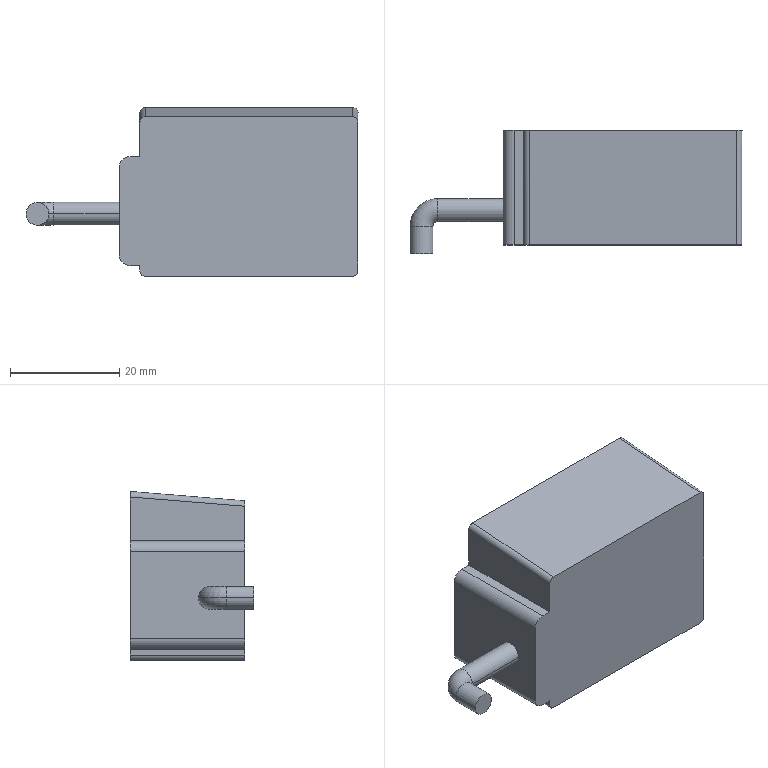Component | SolidWorks | BL-1300-2 | 1 solid | 31 faces | box 60.9 x 22.6 x 31 mm | volume 27093 mm3 | cylinder 14 | plane 11 | cone 4 | torus 2 | commonest cylinder face diameters 4.2 x4 2.5 x4 2 x4 4 x2
build123d program:
from build123d import *

# Parameters (mm, degrees)
BOSS_EXTRUDE1_DEPTH   = 20
M3_TAPPED_HOLE1_D     = 2.5
M3_TAPPED_HOLE1_DEPTH = 7.5
M3_TAPPED_HOLE1_TIP   = 0.7511
SKETCH7_W             = 20
SKETCH7_H             = 3.8
BOSS_EXTRUDE3_DEPTH   = 21
SKETCH8_R             = 2.1
FILLET1_R             = 2
FILLET2_R             = 1


with BuildPart() as part:
    # Sketch2 → Boss-Extrude1 (new, symmetric)
    with BuildSketch(Plane.XY):
        Polygon((0, 0), (31, 0), (29.3, 21), (0, 21), align=None)
    extrude(amount=BOSS_EXTRUDE1_DEPTH, both=True)

    # M3 Tapped Hole1
    with Locations(Plane(origin=(0, 0, 0), x_dir=(-1, 0, 0), z_dir=(0, -1, 0))):
        with Locations((-3.5, -16.5), (-26, 16.5)):
            Hole(M3_TAPPED_HOLE1_D / 2, depth=M3_TAPPED_HOLE1_DEPTH)
            with Locations((0, 0, -(M3_TAPPED_HOLE1_DEPTH + M3_TAPPED_HOLE1_TIP / 2))):  # 118° drill point
                Cone(0, M3_TAPPED_HOLE1_D / 2, M3_TAPPED_HOLE1_TIP, mode=Mode.SUBTRACT)

    # Sketch7 → Boss-Extrude3 (add)
    with BuildSketch(Plane.XZ):
        with Locations((12, -21.9)):
            Rectangle(SKETCH7_W, SKETCH7_H)
    extrude(amount=-BOSS_EXTRUDE3_DEPTH)

    # Sweep1: sweep along a path in Sketch9
    with BuildLine(Plane.ZY.offset(-11.5)) as sweep1_path:
        Line((-23.8, 14.6), (-35.8, 14.6))
        ThreePointArc((-35.8, 14.6), (-37.921, 15.479), (-38.8, 17.6))
        Line((-38.8, 17.6), (-38.8, 22.6))
    # Sketch8 → Sweep1 (sweep)
    with BuildSketch(Plane(origin=(0, 0, -23.8), x_dir=(-1, 0, 0), z_dir=(0, 0, -1))):
        with Locations((-11.5, 14.6)):
            Circle(SKETCH8_R)
    sweep(path=sweep1_path.line)

    # Fillet1
    fillet1_edges = [part.edges().sort_by_distance(p)[0] for p in [
        (22, 10.5, -23.8),
        (2, 10.5, -23.8),
    ]]
    fillet(fillet1_edges, radius=FILLET1_R)

    # Fillet2
    fillet2_edges = [part.edges().sort_by_distance(p)[0] for p in [
        (30.15, 10.5, 20),
        (30.15, 10.5, -20),
        (0, 10.5, -20),
        (0, 10.5, 20),
    ]]
    fillet(fillet2_edges, radius=FILLET2_R)


solid = part.part

# Placed as in the assembly
solid = solid.moved(Location((-14.281, -110.523, -276.479), (180, 90, 0)))
STEP:
#1=CARTESIAN_POINT('',(-1.972,-5.009,-10.432));
#2=VERTEX_POINT('',#1);
#3=CARTESIAN_POINT('',(-1.972,-4.843,-10.432));
#4=VERTEX_POINT('',#3);
#5=CARTESIAN_POINT('',(-1.972,-4.926,-10.432));
#6=DIRECTION('',(-1.,-0.,0.));
#7=DIRECTION('',(-0.,0.,-1.));
#8=AXIS2_PLACEMENT_3D('',#5,#6,#7);
#9=CIRCLE('',#8,0.08268);
#10=EDGE_CURVE('',#2,#4,#9,.T.);
#11=ORIENTED_EDGE('',*,*,#10,.T.);
#12=CARTESIAN_POINT('',(-2.172,-5.044,-10.432));
#13=VERTEX_POINT('',#12);
#14=CARTESIAN_POINT('',(-1.972,-5.044,-10.432));
#15=DIRECTION('',(0.,0.,1.));
#16=DIRECTION('',(1.,0.,-0.));
#17=AXIS2_PLACEMENT_3D('',#14,#15,#16);
#18=CIRCLE('',#17,0.2008);
#19=EDGE_CURVE('',#4,#13,#18,.T.);
#20=ORIENTED_EDGE('',*,*,#19,.T.);
#21=CARTESIAN_POINT('',(-2.007,-5.044,-10.432));
#22=VERTEX_POINT('',#21);
#23=CARTESIAN_POINT('',(-2.09,-5.044,-10.432));
#24=DIRECTION('',(0.,-1.,0.));
#25=DIRECTION('',(-0.,0.,-1.));
#26=AXIS2_PLACEMENT_3D('',#23,#24,#25);
#27=CIRCLE('',#26,0.08268);
#28=EDGE_CURVE('',#22,#13,#27,.T.);
#29=ORIENTED_EDGE('',*,*,#28,.F.);
#30=CARTESIAN_POINT('',(-1.972,-5.044,-10.432));
#31=DIRECTION('',(0.,0.,1.));
#32=DIRECTION('',(1.,0.,-0.));
#33=AXIS2_PLACEMENT_3D('',#30,#31,#32);
#34=CIRCLE('',#33,0.03543);
#35=EDGE_CURVE('',#2,#22,#34,.T.);
#36=ORIENTED_EDGE('',*,*,#35,.F.);
#37=EDGE_LOOP('',(#11,#20,#29,#36));
#38=FACE_OUTER_BOUND('',#37,.T.);
#39=CARTESIAN_POINT('',(-1.972,-5.044,-10.432));
#40=DIRECTION('',(0.,0.,1.));
#41=DIRECTION('',(0.,-1.,0.));
#42=AXIS2_PLACEMENT_3D('',#39,#40,#41);
#43=TOROIDAL_SURFACE('',#42,0.1181,0.08268);
#44=ADVANCED_FACE('',(#38),#43,.T.);
#45=ORIENTED_EDGE('',*,*,#10,.F.);
#46=CARTESIAN_POINT('',(-1.499,-5.009,-10.432));
#47=VERTEX_POINT('',#46);
#48=CARTESIAN_POINT('',(-1.972,-5.009,-10.432));
#49=DIRECTION('',(1.,0.,-0.));
#50=VECTOR('',#49,39.37);
#51=LINE('',#48,#50);
#52=EDGE_CURVE('',#2,#47,#51,.T.);
#53=ORIENTED_EDGE('',*,*,#52,.T.);
#54=CARTESIAN_POINT('',(-1.499,-4.843,-10.432));
#55=VERTEX_POINT('',#54);
#56=CARTESIAN_POINT('',(-1.499,-4.926,-10.432));
#57=DIRECTION('',(-1.,-0.,0.));
#58=DIRECTION('',(-0.,0.,-1.));
#59=AXIS2_PLACEMENT_3D('',#56,#57,#58);
#60=CIRCLE('',#59,0.08268);
#61=EDGE_CURVE('',#47,#55,#60,.T.);
#62=ORIENTED_EDGE('',*,*,#61,.T.);
#63=CARTESIAN_POINT('',(-1.972,-4.843,-10.432));
#64=DIRECTION('',(1.,0.,-0.));
#65=VECTOR('',#64,39.37);
#66=LINE('',#63,#65);
#67=EDGE_CURVE('',#4,#55,#66,.T.);
#68=ORIENTED_EDGE('',*,*,#67,.F.);
#69=EDGE_LOOP('',(#45,#53,#62,#68));
#70=FACE_OUTER_BOUND('',#69,.T.);
#71=CARTESIAN_POINT('',(-1.972,-4.926,-10.432));
#72=DIRECTION('',(1.,0.,-0.));
#73=DIRECTION('',(0.,1.,0.));
#74=AXIS2_PLACEMENT_3D('',#71,#72,#73);
#75=CYLINDRICAL_SURFACE('',#74,0.08268);
#76=ADVANCED_FACE('',(#70),#75,.T.);
#77=ORIENTED_EDGE('',*,*,#28,.T.);
#78=CARTESIAN_POINT('',(-2.172,-5.241,-10.432));
#79=VERTEX_POINT('',#78);
#80=CARTESIAN_POINT('',(-2.172,-5.044,-10.432));
#81=DIRECTION('',(0.,-1.,0.));
#82=VECTOR('',#81,39.37);
#83=LINE('',#80,#82);
#84=EDGE_CURVE('',#13,#79,#83,.T.);
#85=ORIENTED_EDGE('',*,*,#84,.T.);
#86=CARTESIAN_POINT('',(-2.007,-5.241,-10.432));
#87=VERTEX_POINT('',#86);
#88=CARTESIAN_POINT('',(-2.09,-5.241,-10.432));
#89=DIRECTION('',(0.,-1.,0.));
#90=DIRECTION('',(-0.,0.,-1.));
#91=AXIS2_PLACEMENT_3D('',#88,#89,#90);
#92=CIRCLE('',#91,0.08268);
#93=EDGE_CURVE('',#87,#79,#92,.T.);
#94=ORIENTED_EDGE('',*,*,#93,.F.);
#95=CARTESIAN_POINT('',(-2.007,-5.044,-10.432));
#96=DIRECTION('',(0.,-1.,0.));
#97=VECTOR('',#96,39.37);
#98=LINE('',#95,#97);
#99=EDGE_CURVE('',#22,#87,#98,.T.);
#100=ORIENTED_EDGE('',*,*,#99,.F.);
#101=EDGE_LOOP('',(#77,#85,#94,#100));
#102=FACE_OUTER_BOUND('',#101,.T.);
#103=CARTESIAN_POINT('',(-2.09,-5.044,-10.432));
#104=DIRECTION('',(0.,-1.,0.));
#105=DIRECTION('',(1.,0.,-0.));
#106=AXIS2_PLACEMENT_3D('',#103,#104,#105);
#107=CYLINDRICAL_SURFACE('',#106,0.08268);
#108=ADVANCED_FACE('',(#102),#107,.T.);
#109=CARTESIAN_POINT('',(0.1366,-4.647,-10.747));
#110=VERTEX_POINT('',#109);
#111=CARTESIAN_POINT('',(0.03816,-4.647,-10.747));
#112=VERTEX_POINT('',#111);
#113=CARTESIAN_POINT('',(0.08738,-4.647,-10.747));
#114=DIRECTION('',(-0.,1.,-0.));
#115=DIRECTION('',(-1.,0.,0.));
#116=AXIS2_PLACEMENT_3D('',#113,#114,#115);
#117=CIRCLE('',#116,0.04921);
#118=EDGE_CURVE('',#110,#112,#117,.T.);
#119=ORIENTED_EDGE('',*,*,#118,.F.);
#120=CARTESIAN_POINT('',(0.1366,-4.351,-10.747));
#121=VERTEX_POINT('',#120);
#122=CARTESIAN_POINT('',(0.1366,-4.351,-10.747));
#123=DIRECTION('',(-0.,1.,-0.));
#124=VECTOR('',#123,39.37);
#125=LINE('',#122,#124);
#126=EDGE_CURVE('',#110,#121,#125,.T.);
#127=ORIENTED_EDGE('',*,*,#126,.T.);
#128=CARTESIAN_POINT('',(0.03816,-4.351,-10.747));
#129=VERTEX_POINT('',#128);
#130=CARTESIAN_POINT('',(0.08738,-4.351,-10.747));
#131=DIRECTION('',(-0.,1.,-0.));
#132=DIRECTION('',(-1.,0.,0.));
#133=AXIS2_PLACEMENT_3D('',#130,#131,#132);
#134=CIRCLE('',#133,0.04921);
#135=EDGE_CURVE('',#121,#129,#134,.T.);
#136=ORIENTED_EDGE('',*,*,#135,.T.);
#137=CARTESIAN_POINT('',(0.03816,-4.351,-10.747));
#138=DIRECTION('',(-0.,1.,-0.));
#139=VECTOR('',#138,39.37);
#140=LINE('',#137,#139);
#141=EDGE_CURVE('',#112,#129,#140,.T.);
#142=ORIENTED_EDGE('',*,*,#141,.F.);
#143=EDGE_LOOP('',(#119,#127,#136,#142));
#144=FACE_OUTER_BOUND('',#143,.T.);
#145=CARTESIAN_POINT('',(0.08738,-4.351,-10.747));
#146=DIRECTION('',(-0.,1.,-0.));
#147=DIRECTION('',(-1.,0.,0.));
#148=AXIS2_PLACEMENT_3D('',#145,#146,#147);
#149=CYLINDRICAL_SURFACE('',#148,0.04921);
#150=ADVANCED_FACE('',(#144),#149,.F.);
#151=CARTESIAN_POINT('',(0.08738,-4.676,-10.747));
#152=VERTEX_POINT('',#151);
#153=CARTESIAN_POINT('',(0.03816,-4.647,-10.747));
#154=DIRECTION('',(-0.8572,0.515,0.));
#155=VECTOR('',#154,39.37);
#156=LINE('',#153,#155);
#157=EDGE_CURVE('',#152,#112,#156,.T.);
#158=ORIENTED_EDGE('',*,*,#157,.F.);
#159=CARTESIAN_POINT('',(0.1366,-4.647,-10.747));
#160=DIRECTION('',(0.8572,0.515,-0.));
#161=VECTOR('',#160,39.37);
#162=LINE('',#159,#161);
#163=EDGE_CURVE('',#152,#110,#162,.T.);
#164=ORIENTED_EDGE('',*,*,#163,.T.);
#165=ORIENTED_EDGE('',*,*,#118,.T.);
#166=EDGE_LOOP('',(#158,#164,#165));
#167=FACE_OUTER_BOUND('',#166,.T.);
#168=CARTESIAN_POINT('',(0.08738,-4.647,-10.747));
#169=DIRECTION('',(-0.,1.,-0.));
#170=DIRECTION('',(-1.,0.,0.));
#171=AXIS2_PLACEMENT_3D('',#168,#169,#170);
#172=CONICAL_SURFACE('',#171,0.04921,1.03);
#173=ADVANCED_FACE('',(#167),#172,.F.);
#174=CARTESIAN_POINT('',(-1.163,-4.647,-9.861));
#175=VERTEX_POINT('',#174);
#176=CARTESIAN_POINT('',(-1.261,-4.647,-9.861));
#177=VERTEX_POINT('',#176);
#178=CARTESIAN_POINT('',(-1.212,-4.647,-9.861));
#179=DIRECTION('',(-0.,1.,-0.));
#180=DIRECTION('',(-1.,0.,0.));
#181=AXIS2_PLACEMENT_3D('',#178,#179,#180);
#182=CIRCLE('',#181,0.04921);
#183=EDGE_CURVE('',#175,#177,#182,.T.);
#184=ORIENTED_EDGE('',*,*,#183,.F.);
#185=CARTESIAN_POINT('',(-1.163,-4.351,-9.861));
#186=VERTEX_POINT('',#185);
#187=CARTESIAN_POINT('',(-1.163,-4.351,-9.861));
#188=DIRECTION('',(-0.,1.,-0.));
#189=VECTOR('',#188,39.37);
#190=LINE('',#187,#189);
#191=EDGE_CURVE('',#175,#186,#190,.T.);
#192=ORIENTED_EDGE('',*,*,#191,.T.);
#193=CARTESIAN_POINT('',(-1.261,-4.351,-9.861));
#194=VERTEX_POINT('',#193);
#195=CARTESIAN_POINT('',(-1.212,-4.351,-9.861));
#196=DIRECTION('',(-0.,1.,-0.));
#197=DIRECTION('',(-1.,0.,0.));
#198=AXIS2_PLACEMENT_3D('',#195,#196,#197);
#199=CIRCLE('',#198,0.04921);
#200=EDGE_CURVE('',#186,#194,#199,.T.);
#201=ORIENTED_EDGE('',*,*,#200,.T.);
#202=CARTESIAN_POINT('',(-1.261,-4.351,-9.861));
#203=DIRECTION('',(-0.,1.,-0.));
#204=VECTOR('',#203,39.37);
#205=LINE('',#202,#204);
#206=EDGE_CURVE('',#177,#194,#205,.T.);
#207=ORIENTED_EDGE('',*,*,#206,.F.);
#208=EDGE_LOOP('',(#184,#192,#201,#207));
#209=FACE_OUTER_BOUND('',#208,.T.);
#210=CARTESIAN_POINT('',(-1.212,-4.351,-9.861));
#211=DIRECTION('',(-0.,1.,-0.));
#212=DIRECTION('',(-1.,0.,0.));
#213=AXIS2_PLACEMENT_3D('',#210,#211,#212);
#214=CYLINDRICAL_SURFACE('',#213,0.04921);
#215=ADVANCED_FACE('',(#209),#214,.F.);
#216=CARTESIAN_POINT('',(-1.212,-4.676,-9.861));
#217=VERTEX_POINT('',#216);
#218=CARTESIAN_POINT('',(-1.261,-4.647,-9.861));
#219=DIRECTION('',(-0.8572,0.515,0.));
#220=VECTOR('',#219,39.37);
#221=LINE('',#218,#220);
#222=EDGE_CURVE('',#217,#177,#221,.T.);
#223=ORIENTED_EDGE('',*,*,#222,.F.);
#224=CARTESIAN_POINT('',(-1.163,-4.647,-9.861));
#225=DIRECTION('',(0.8572,0.515,-0.));
#226=VECTOR('',#225,39.37);
#227=LINE('',#224,#226);
#228=EDGE_CURVE('',#217,#175,#227,.T.);
#229=ORIENTED_EDGE('',*,*,#228,.T.);
#230=ORIENTED_EDGE('',*,*,#183,.T.);
#231=EDGE_LOOP('',(#223,#229,#230));
#232=FACE_OUTER_BOUND('',#231,.T.);
#233=CARTESIAN_POINT('',(-1.212,-4.647,-9.861));
#234=DIRECTION('',(-0.,1.,-0.));
#235=DIRECTION('',(-1.,0.,0.));
#236=AXIS2_PLACEMENT_3D('',#233,#234,#235);
#237=CONICAL_SURFACE('',#236,0.04921,1.03);
#238=ADVANCED_FACE('',(#232),#237,.F.);
#239=CARTESIAN_POINT('',(-1.35,-5.178,-9.771));
#240=VERTEX_POINT('',#239);
#241=CARTESIAN_POINT('',(-1.35,-5.178,-10.019));
#242=VERTEX_POINT('',#241);
#243=CARTESIAN_POINT('',(-1.35,-5.178,-9.731));
#244=DIRECTION('',(-0.,-0.,-1.));
#245=VECTOR('',#244,39.37);
#246=LINE('',#243,#245);
#247=EDGE_CURVE('',#240,#242,#246,.T.);
#248=ORIENTED_EDGE('',*,*,#247,.F.);
#249=CARTESIAN_POINT('',(-1.35,-4.351,-9.704));
#250=VERTEX_POINT('',#249);
#251=CARTESIAN_POINT('',(-1.35,-4.446,-9.712));
#252=DIRECTION('',(0.,0.9967,0.08069));
#253=VECTOR('',#252,39.37);
#254=LINE('',#251,#253);
#255=EDGE_CURVE('',#240,#250,#254,.T.);
#256=ORIENTED_EDGE('',*,*,#255,.T.);
#257=CARTESIAN_POINT('',(-1.35,-4.351,-10.019));
#258=VERTEX_POINT('',#257);
#259=CARTESIAN_POINT('',(-1.35,-4.351,-10.885));
#260=DIRECTION('',(0.,0.,1.));
#261=VECTOR('',#260,39.37);
#262=LINE('',#259,#261);
#263=EDGE_CURVE('',#258,#250,#262,.T.);
#264=ORIENTED_EDGE('',*,*,#263,.F.);
#265=CARTESIAN_POINT('',(-1.35,-5.98,-10.019));
#266=DIRECTION('',(-0.,1.,-0.));
#267=VECTOR('',#266,39.37);
#268=LINE('',#265,#267);
#269=EDGE_CURVE('',#242,#258,#268,.T.);
#270=ORIENTED_EDGE('',*,*,#269,.F.);
#271=EDGE_LOOP('',(#248,#256,#264,#270));
#272=FACE_OUTER_BOUND('',#271,.T.);
#273=CARTESIAN_POINT('',(-1.35,-4.351,-10.885));
#274=DIRECTION('',(1.,0.,-0.));
#275=DIRECTION('',(0.,0.,1.));
#276=AXIS2_PLACEMENT_3D('',#273,#274,#275);
#277=PLANE('',#276);
#278=ADVANCED_FACE('',(#272),#277,.F.);
#279=CARTESIAN_POINT('',(0.1858,-5.178,-10.885));
#280=VERTEX_POINT('',#279);
#281=CARTESIAN_POINT('',(-1.31,-5.178,-10.885));
#282=VERTEX_POINT('',#281);
#283=CARTESIAN_POINT('',(0.2252,-5.178,-10.885));
#284=DIRECTION('',(-1.,-0.,0.));
#285=VECTOR('',#284,39.37);
#286=LINE('',#283,#285);
#287=EDGE_CURVE('',#280,#282,#286,.T.);
#288=ORIENTED_EDGE('',*,*,#287,.T.);
#289=CARTESIAN_POINT('',(-1.31,-4.351,-10.885));
#290=VERTEX_POINT('',#289);
#291=CARTESIAN_POINT('',(-1.31,-5.178,-10.885));
#292=DIRECTION('',(-0.,1.,-0.));
#293=VECTOR('',#292,39.37);
#294=LINE('',#291,#293);
#295=EDGE_CURVE('',#282,#290,#294,.T.);
#296=ORIENTED_EDGE('',*,*,#295,.T.);
#297=CARTESIAN_POINT('',(0.1858,-4.351,-10.885));
#298=VERTEX_POINT('',#297);
#299=CARTESIAN_POINT('',(0.2252,-4.351,-10.885));
#300=DIRECTION('',(-1.,-0.,0.));
#301=VECTOR('',#300,39.37);
#302=LINE('',#299,#301);
#303=EDGE_CURVE('',#298,#290,#302,.T.);
#304=ORIENTED_EDGE('',*,*,#303,.F.);
#305=CARTESIAN_POINT('',(0.1858,-5.178,-10.885));
#306=DIRECTION('',(0.,-1.,0.));
#307=VECTOR('',#306,39.37);
#308=LINE('',#305,#307);
#309=EDGE_CURVE('',#298,#280,#308,.T.);
#310=ORIENTED_EDGE('',*,*,#309,.T.);
#311=EDGE_LOOP('',(#288,#296,#304,#310));
#312=FACE_OUTER_BOUND('',#311,.T.);
#313=CARTESIAN_POINT('',(0.2252,-5.178,-10.885));
#314=DIRECTION('',(0.,0.,1.));
#315=DIRECTION('',(0.,-1.,0.));
#316=AXIS2_PLACEMENT_3D('',#313,#314,#315);
#317=PLANE('',#316);
#318=ADVANCED_FACE('',(#312),#317,.F.);
#319=CARTESIAN_POINT('',(0.08738,-4.351,-10.747));
#320=DIRECTION('',(-0.,1.,-0.));
#321=DIRECTION('',(-1.,0.,0.));
#322=AXIS2_PLACEMENT_3D('',#319,#320,#321);
#323=CIRCLE('',#322,0.04921);
#324=EDGE_CURVE('',#129,#121,#323,.T.);
#325=ORIENTED_EDGE('',*,*,#324,.F.);
#326=ORIENTED_EDGE('',*,*,#135,.F.);
#327=EDGE_LOOP('',(#325,#326));
#328=FACE_BOUND('',#327,.T.);
#329=CARTESIAN_POINT('',(-1.212,-4.351,-9.861));
#330=DIRECTION('',(-0.,1.,-0.));
#331=DIRECTION('',(-1.,0.,0.));
#332=AXIS2_PLACEMENT_3D('',#329,#330,#331);
#333=CIRCLE('',#332,0.04921);
#334=EDGE_CURVE('',#194,#186,#333,.T.);
#335=ORIENTED_EDGE('',*,*,#334,.F.);
#336=ORIENTED_EDGE('',*,*,#200,.F.);
#337=EDGE_LOOP('',(#335,#336));
#338=FACE_BOUND('',#337,.T.);
#339=ORIENTED_EDGE('',*,*,#263,.T.);
#340=CARTESIAN_POINT('',(-1.31,-4.351,-9.665));
#341=VERTEX_POINT('',#340);
#342=CARTESIAN_POINT('',(-1.35,-4.351,-9.704));
#343=CARTESIAN_POINT('',(-1.35,-4.351,-9.681));
#344=CARTESIAN_POINT('',(-1.333,-4.351,-9.665));
#345=CARTESIAN_POINT('',(-1.31,-4.351,-9.665));
#346=(BOUNDED_CURVE()B_SPLINE_CURVE(3,(#342,#343,#344,#345),.UNSPECIFIED.,.F.,.T.)B_SPLINE_CURVE_WITH_KNOTS((4,4),(1.571,3.142),.UNSPECIFIED.)CURVE()GEOMETRIC_REPRESENTATION_ITEM()RATIONAL_B_SPLINE_CURVE((1.,0.8047,0.8047,1.))REPRESENTATION_ITEM(''));
#347=EDGE_CURVE('',#250,#341,#346,.T.);
#348=ORIENTED_EDGE('',*,*,#347,.T.);
#349=CARTESIAN_POINT('',(0.1858,-4.351,-9.665));
#350=VERTEX_POINT('',#349);
#351=CARTESIAN_POINT('',(0.2252,-4.351,-9.665));
#352=DIRECTION('',(-1.,-0.,0.));
#353=VECTOR('',#352,39.37);
#354=LINE('',#351,#353);
#355=EDGE_CURVE('',#350,#341,#354,.T.);
#356=ORIENTED_EDGE('',*,*,#355,.F.);
#357=CARTESIAN_POINT('',(0.2252,-4.351,-9.704));
#358=VERTEX_POINT('',#357);
#359=CARTESIAN_POINT('',(0.1858,-4.351,-9.665));
#360=CARTESIAN_POINT('',(0.2089,-4.351,-9.665));
#361=CARTESIAN_POINT('',(0.2252,-4.351,-9.681));
#362=CARTESIAN_POINT('',(0.2252,-4.351,-9.704));
#363=(BOUNDED_CURVE()B_SPLINE_CURVE(3,(#359,#360,#361,#362),.UNSPECIFIED.,.F.,.T.)B_SPLINE_CURVE_WITH_KNOTS((4,4),(0.,1.571),.UNSPECIFIED.)CURVE()GEOMETRIC_REPRESENTATION_ITEM()RATIONAL_B_SPLINE_CURVE((1.,0.8047,0.8047,1.))REPRESENTATION_ITEM(''));
#364=EDGE_CURVE('',#350,#358,#363,.T.);
#365=ORIENTED_EDGE('',*,*,#364,.T.);
#366=CARTESIAN_POINT('',(0.2252,-4.351,-10.846));
#367=VERTEX_POINT('',#366);
#368=CARTESIAN_POINT('',(0.2252,-4.351,-10.885));
#369=DIRECTION('',(0.,0.,1.));
#370=VECTOR('',#369,39.37);
#371=LINE('',#368,#370);
#372=EDGE_CURVE('',#367,#358,#371,.T.);
#373=ORIENTED_EDGE('',*,*,#372,.F.);
#374=CARTESIAN_POINT('',(0.1858,-4.351,-10.846));
#375=DIRECTION('',(-0.,1.,-0.));
#376=DIRECTION('',(1.,0.,-0.));
#377=AXIS2_PLACEMENT_3D('',#374,#375,#376);
#378=CIRCLE('',#377,0.03937);
#379=EDGE_CURVE('',#367,#298,#378,.T.);
#380=ORIENTED_EDGE('',*,*,#379,.T.);
#381=ORIENTED_EDGE('',*,*,#303,.T.);
#382=CARTESIAN_POINT('',(-1.35,-4.351,-10.846));
#383=VERTEX_POINT('',#382);
#384=CARTESIAN_POINT('',(-1.31,-4.351,-10.846));
#385=DIRECTION('',(-0.,1.,-0.));
#386=DIRECTION('',(1.,0.,-0.));
#387=AXIS2_PLACEMENT_3D('',#384,#385,#386);
#388=CIRCLE('',#387,0.03937);
#389=EDGE_CURVE('',#290,#383,#388,.T.);
#390=ORIENTED_EDGE('',*,*,#389,.T.);
#391=CARTESIAN_POINT('',(-1.35,-4.351,-10.806));
#392=VERTEX_POINT('',#391);
#393=CARTESIAN_POINT('',(-1.35,-4.351,-10.885));
#394=DIRECTION('',(0.,0.,1.));
#395=VECTOR('',#394,39.37);
#396=LINE('',#393,#395);
#397=EDGE_CURVE('',#383,#392,#396,.T.);
#398=ORIENTED_EDGE('',*,*,#397,.T.);
#399=CARTESIAN_POINT('',(-1.42,-4.351,-10.806));
#400=VERTEX_POINT('',#399);
#401=CARTESIAN_POINT('',(-1.35,-4.351,-10.806));
#402=DIRECTION('',(-1.,-0.,0.));
#403=VECTOR('',#402,39.37);
#404=LINE('',#401,#403);
#405=EDGE_CURVE('',#392,#400,#404,.T.);
#406=ORIENTED_EDGE('',*,*,#405,.T.);
#407=CARTESIAN_POINT('',(-1.499,-4.351,-10.728));
#408=VERTEX_POINT('',#407);
#409=CARTESIAN_POINT('',(-1.42,-4.351,-10.728));
#410=DIRECTION('',(-0.,1.,-0.));
#411=DIRECTION('',(1.,0.,-0.));
#412=AXIS2_PLACEMENT_3D('',#409,#410,#411);
#413=CIRCLE('',#412,0.07874);
#414=EDGE_CURVE('',#400,#408,#413,.T.);
#415=ORIENTED_EDGE('',*,*,#414,.T.);
#416=CARTESIAN_POINT('',(-1.499,-4.351,-10.098));
#417=VERTEX_POINT('',#416);
#418=CARTESIAN_POINT('',(-1.499,-4.351,-10.806));
#419=DIRECTION('',(0.,0.,1.));
#420=VECTOR('',#419,39.37);
#421=LINE('',#418,#420);
#422=EDGE_CURVE('',#408,#417,#421,.T.);
#423=ORIENTED_EDGE('',*,*,#422,.T.);
#424=CARTESIAN_POINT('',(-1.42,-4.351,-10.019));
#425=VERTEX_POINT('',#424);
#426=CARTESIAN_POINT('',(-1.42,-4.351,-10.098));
#427=DIRECTION('',(-0.,1.,-0.));
#428=DIRECTION('',(1.,0.,-0.));
#429=AXIS2_PLACEMENT_3D('',#426,#427,#428);
#430=CIRCLE('',#429,0.07874);
#431=EDGE_CURVE('',#417,#425,#430,.T.);
#432=ORIENTED_EDGE('',*,*,#431,.T.);
#433=CARTESIAN_POINT('',(-1.35,-4.351,-10.019));
#434=DIRECTION('',(1.,0.,-0.));
#435=VECTOR('',#434,39.37);
#436=LINE('',#433,#435);
#437=EDGE_CURVE('',#425,#258,#436,.T.);
#438=ORIENTED_EDGE('',*,*,#437,.T.);
#439=EDGE_LOOP('',(#339,#348,#356,#365,#373,#380,#381,#390,#398,#406,#415,#423,#432,#438));
#440=FACE_OUTER_BOUND('',#439,.T.);
#441=CARTESIAN_POINT('',(0.2252,-4.351,-10.885));
#442=DIRECTION('',(0.,-1.,0.));
#443=DIRECTION('',(1.,0.,-0.));
#444=AXIS2_PLACEMENT_3D('',#441,#442,#443);
#445=PLANE('',#444);
#446=ADVANCED_FACE('',(#328,#338,#440),#445,.F.);
#447=ORIENTED_EDGE('',*,*,#355,.T.);
#448=CARTESIAN_POINT('',(-1.31,-5.178,-9.731));
#449=VERTEX_POINT('',#448);
#450=CARTESIAN_POINT('',(-1.31,-4.351,-9.665));
#451=DIRECTION('',(-0.,-0.9967,-0.08069));
#452=VECTOR('',#451,39.37);
#453=LINE('',#450,#452);
#454=EDGE_CURVE('',#341,#449,#453,.T.);
#455=ORIENTED_EDGE('',*,*,#454,.T.);
#456=CARTESIAN_POINT('',(0.1858,-5.178,-9.731));
#457=VERTEX_POINT('',#456);
#458=CARTESIAN_POINT('',(0.2252,-5.178,-9.731));
#459=DIRECTION('',(-1.,-0.,0.));
#460=VECTOR('',#459,39.37);
#461=LINE('',#458,#460);
#462=EDGE_CURVE('',#457,#449,#461,.T.);
#463=ORIENTED_EDGE('',*,*,#462,.F.);
#464=CARTESIAN_POINT('',(0.1858,-4.351,-9.665));
#465=DIRECTION('',(0.,0.9967,0.08069));
#466=VECTOR('',#465,39.37);
#467=LINE('',#464,#466);
#468=EDGE_CURVE('',#457,#350,#467,.T.);
#469=ORIENTED_EDGE('',*,*,#468,.T.);
#470=EDGE_LOOP('',(#447,#455,#463,#469));
#471=FACE_OUTER_BOUND('',#470,.T.);
#472=CARTESIAN_POINT('',(0.2252,-4.351,-9.665));
#473=DIRECTION('',(-0.,0.08069,-0.9967));
#474=DIRECTION('',(0.,0.9967,0.08069));
#475=AXIS2_PLACEMENT_3D('',#472,#473,#474);
#476=PLANE('',#475);
#477=ADVANCED_FACE('',(#471),#476,.F.);
#478=ORIENTED_EDGE('',*,*,#462,.T.);
#479=CARTESIAN_POINT('',(-1.31,-5.178,-9.731));
#480=CARTESIAN_POINT('',(-1.333,-5.178,-9.731));
#481=CARTESIAN_POINT('',(-1.35,-5.178,-9.748));
#482=CARTESIAN_POINT('',(-1.35,-5.178,-9.771));
#483=(BOUNDED_CURVE()B_SPLINE_CURVE(3,(#479,#480,#481,#482),.UNSPECIFIED.,.F.,.T.)B_SPLINE_CURVE_WITH_KNOTS((4,4),(3.142,4.712),.UNSPECIFIED.)CURVE()GEOMETRIC_REPRESENTATION_ITEM()RATIONAL_B_SPLINE_CURVE((1.,0.8047,0.8047,1.))REPRESENTATION_ITEM(''));
#484=EDGE_CURVE('',#449,#240,#483,.T.);
#485=ORIENTED_EDGE('',*,*,#484,.T.);
#486=ORIENTED_EDGE('',*,*,#247,.T.);
#487=CARTESIAN_POINT('',(-1.42,-5.178,-10.019));
#488=VERTEX_POINT('',#487);
#489=CARTESIAN_POINT('',(-1.35,-5.178,-10.019));
#490=DIRECTION('',(-1.,-0.,0.));
#491=VECTOR('',#490,39.37);
#492=LINE('',#489,#491);
#493=EDGE_CURVE('',#242,#488,#492,.T.);
#494=ORIENTED_EDGE('',*,*,#493,.T.);
#495=CARTESIAN_POINT('',(-1.499,-5.178,-10.098));
#496=VERTEX_POINT('',#495);
#497=CARTESIAN_POINT('',(-1.42,-5.178,-10.098));
#498=DIRECTION('',(0.,-1.,0.));
#499=DIRECTION('',(0.,0.,1.));
#500=AXIS2_PLACEMENT_3D('',#497,#498,#499);
#501=CIRCLE('',#500,0.07874);
#502=EDGE_CURVE('',#488,#496,#501,.T.);
#503=ORIENTED_EDGE('',*,*,#502,.T.);
#504=CARTESIAN_POINT('',(-1.499,-5.178,-10.728));
#505=VERTEX_POINT('',#504);
#506=CARTESIAN_POINT('',(-1.499,-5.178,-10.806));
#507=DIRECTION('',(-0.,-0.,-1.));
#508=VECTOR('',#507,39.37);
#509=LINE('',#506,#508);
#510=EDGE_CURVE('',#496,#505,#509,.T.);
#511=ORIENTED_EDGE('',*,*,#510,.T.);
#512=CARTESIAN_POINT('',(-1.42,-5.178,-10.806));
#513=VERTEX_POINT('',#512);
#514=CARTESIAN_POINT('',(-1.42,-5.178,-10.728));
#515=DIRECTION('',(0.,-1.,0.));
#516=DIRECTION('',(0.,0.,1.));
#517=AXIS2_PLACEMENT_3D('',#514,#515,#516);
#518=CIRCLE('',#517,0.07874);
#519=EDGE_CURVE('',#505,#513,#518,.T.);
#520=ORIENTED_EDGE('',*,*,#519,.T.);
#521=CARTESIAN_POINT('',(-1.35,-5.178,-10.806));
#522=VERTEX_POINT('',#521);
#523=CARTESIAN_POINT('',(-1.35,-5.178,-10.806));
#524=DIRECTION('',(1.,0.,-0.));
#525=VECTOR('',#524,39.37);
#526=LINE('',#523,#525);
#527=EDGE_CURVE('',#513,#522,#526,.T.);
#528=ORIENTED_EDGE('',*,*,#527,.T.);
#529=CARTESIAN_POINT('',(-1.35,-5.178,-10.846));
#530=VERTEX_POINT('',#529);
#531=CARTESIAN_POINT('',(-1.35,-5.178,-9.731));
#532=DIRECTION('',(-0.,-0.,-1.));
#533=VECTOR('',#532,39.37);
#534=LINE('',#531,#533);
#535=EDGE_CURVE('',#522,#530,#534,.T.);
#536=ORIENTED_EDGE('',*,*,#535,.T.);
#537=CARTESIAN_POINT('',(-1.31,-5.178,-10.846));
#538=DIRECTION('',(0.,-1.,0.));
#539=DIRECTION('',(0.,0.,1.));
#540=AXIS2_PLACEMENT_3D('',#537,#538,#539);
#541=CIRCLE('',#540,0.03937);
#542=EDGE_CURVE('',#530,#282,#541,.T.);
#543=ORIENTED_EDGE('',*,*,#542,.T.);
#544=ORIENTED_EDGE('',*,*,#287,.F.);
#545=CARTESIAN_POINT('',(0.2252,-5.178,-10.846));
#546=VERTEX_POINT('',#545);
#547=CARTESIAN_POINT('',(0.1858,-5.178,-10.846));
#548=DIRECTION('',(0.,-1.,0.));
#549=DIRECTION('',(0.,0.,1.));
#550=AXIS2_PLACEMENT_3D('',#547,#548,#549);
#551=CIRCLE('',#550,0.03937);
#552=EDGE_CURVE('',#280,#546,#551,.T.);
#553=ORIENTED_EDGE('',*,*,#552,.T.);
#554=CARTESIAN_POINT('',(0.2252,-5.178,-9.771));
#555=VERTEX_POINT('',#554);
#556=CARTESIAN_POINT('',(0.2252,-5.178,-9.731));
#557=DIRECTION('',(-0.,-0.,-1.));
#558=VECTOR('',#557,39.37);
#559=LINE('',#556,#558);
#560=EDGE_CURVE('',#555,#546,#559,.T.);
#561=ORIENTED_EDGE('',*,*,#560,.F.);
#562=CARTESIAN_POINT('',(0.2252,-5.178,-9.771));
#563=CARTESIAN_POINT('',(0.2252,-5.178,-9.748));
#564=CARTESIAN_POINT('',(0.2089,-5.178,-9.731));
#565=CARTESIAN_POINT('',(0.1858,-5.178,-9.731));
#566=(BOUNDED_CURVE()B_SPLINE_CURVE(3,(#562,#563,#564,#565),.UNSPECIFIED.,.F.,.T.)B_SPLINE_CURVE_WITH_KNOTS((4,4),(4.712,6.283),.UNSPECIFIED.)CURVE()GEOMETRIC_REPRESENTATION_ITEM()RATIONAL_B_SPLINE_CURVE((1.,0.8047,0.8047,1.))REPRESENTATION_ITEM(''));
#567=EDGE_CURVE('',#555,#457,#566,.T.);
#568=ORIENTED_EDGE('',*,*,#567,.T.);
#569=EDGE_LOOP('',(#478,#485,#486,#494,#503,#511,#520,#528,#536,#543,#544,#553,#561,#568));
#570=FACE_OUTER_BOUND('',#569,.T.);
#571=CARTESIAN_POINT('',(0.2252,-5.178,-9.731));
#572=DIRECTION('',(-0.,1.,-0.));
#573=DIRECTION('',(0.,0.,1.));
#574=AXIS2_PLACEMENT_3D('',#571,#572,#573);
#575=PLANE('',#574);
#576=ADVANCED_FACE('',(#570),#575,.F.);
#577=ORIENTED_EDGE('',*,*,#560,.T.);
#578=CARTESIAN_POINT('',(0.2252,-4.351,-10.846));
#579=DIRECTION('',(-0.,1.,-0.));
#580=VECTOR('',#579,39.37);
#581=LINE('',#578,#580);
#582=EDGE_CURVE('',#546,#367,#581,.T.);
#583=ORIENTED_EDGE('',*,*,#582,.T.);
#584=ORIENTED_EDGE('',*,*,#372,.T.);
#585=CARTESIAN_POINT('',(0.2252,-5.175,-9.771));
#586=DIRECTION('',(-0.,-0.9967,-0.08069));
#587=VECTOR('',#586,39.37);
#588=LINE('',#585,#587);
#589=EDGE_CURVE('',#358,#555,#588,.T.);
#590=ORIENTED_EDGE('',*,*,#589,.T.);
#591=EDGE_LOOP('',(#577,#583,#584,#590));
#592=FACE_OUTER_BOUND('',#591,.T.);
#593=CARTESIAN_POINT('',(0.2252,-4.351,-10.885));
#594=DIRECTION('',(1.,0.,-0.));
#595=DIRECTION('',(0.,0.,1.));
#596=AXIS2_PLACEMENT_3D('',#593,#594,#595);
#597=PLANE('',#596);
#598=ADVANCED_FACE('',(#592),#597,.T.);
#599=ORIENTED_EDGE('',*,*,#397,.F.);
#600=CARTESIAN_POINT('',(-1.35,-4.351,-10.846));
#601=DIRECTION('',(0.,-1.,0.));
#602=VECTOR('',#601,39.37);
#603=LINE('',#600,#602);
#604=EDGE_CURVE('',#383,#530,#603,.T.);
#605=ORIENTED_EDGE('',*,*,#604,.T.);
#606=ORIENTED_EDGE('',*,*,#535,.F.);
#607=CARTESIAN_POINT('',(-1.35,-5.98,-10.806));
#608=DIRECTION('',(-0.,1.,-0.));
#609=VECTOR('',#608,39.37);
#610=LINE('',#607,#609);
#611=EDGE_CURVE('',#522,#392,#610,.T.);
#612=ORIENTED_EDGE('',*,*,#611,.T.);
#613=EDGE_LOOP('',(#599,#605,#606,#612));
#614=FACE_OUTER_BOUND('',#613,.T.);
#615=CARTESIAN_POINT('',(-1.35,-4.351,-10.885));
#616=DIRECTION('',(1.,0.,-0.));
#617=DIRECTION('',(0.,0.,1.));
#618=AXIS2_PLACEMENT_3D('',#615,#616,#617);
#619=PLANE('',#618);
#620=ADVANCED_FACE('',(#614),#619,.F.);
#621=ORIENTED_EDGE('',*,*,#228,.F.);
#622=ORIENTED_EDGE('',*,*,#222,.T.);
#623=CARTESIAN_POINT('',(-1.212,-4.647,-9.861));
#624=DIRECTION('',(-0.,1.,-0.));
#625=DIRECTION('',(-1.,0.,0.));
#626=AXIS2_PLACEMENT_3D('',#623,#624,#625);
#627=CIRCLE('',#626,0.04921);
#628=EDGE_CURVE('',#177,#175,#627,.T.);
#629=ORIENTED_EDGE('',*,*,#628,.T.);
#630=EDGE_LOOP('',(#621,#622,#629));
#631=FACE_OUTER_BOUND('',#630,.T.);
#632=CARTESIAN_POINT('',(-1.212,-4.647,-9.861));
#633=DIRECTION('',(-0.,1.,-0.));
#634=DIRECTION('',(-1.,0.,0.));
#635=AXIS2_PLACEMENT_3D('',#632,#633,#634);
#636=CONICAL_SURFACE('',#635,0.04921,1.03);
#637=ADVANCED_FACE('',(#631),#636,.F.);
#638=ORIENTED_EDGE('',*,*,#191,.F.);
#639=ORIENTED_EDGE('',*,*,#628,.F.);
#640=ORIENTED_EDGE('',*,*,#206,.T.);
#641=ORIENTED_EDGE('',*,*,#334,.T.);
#642=EDGE_LOOP('',(#638,#639,#640,#641));
#643=FACE_OUTER_BOUND('',#642,.T.);
#644=CARTESIAN_POINT('',(-1.212,-4.351,-9.861));
#645=DIRECTION('',(-0.,1.,-0.));
#646=DIRECTION('',(-1.,0.,0.));
#647=AXIS2_PLACEMENT_3D('',#644,#645,#646);
#648=CYLINDRICAL_SURFACE('',#647,0.04921);
#649=ADVANCED_FACE('',(#643),#648,.F.);
#650=ORIENTED_EDGE('',*,*,#163,.F.);
#651=ORIENTED_EDGE('',*,*,#157,.T.);
#652=CARTESIAN_POINT('',(0.08738,-4.647,-10.747));
#653=DIRECTION('',(-0.,1.,-0.));
#654=DIRECTION('',(-1.,0.,0.));
#655=AXIS2_PLACEMENT_3D('',#652,#653,#654);
#656=CIRCLE('',#655,0.04921);
#657=EDGE_CURVE('',#112,#110,#656,.T.);
#658=ORIENTED_EDGE('',*,*,#657,.T.);
#659=EDGE_LOOP('',(#650,#651,#658));
#660=FACE_OUTER_BOUND('',#659,.T.);
#661=CARTESIAN_POINT('',(0.08738,-4.647,-10.747));
#662=DIRECTION('',(-0.,1.,-0.));
#663=DIRECTION('',(-1.,0.,0.));
#664=AXIS2_PLACEMENT_3D('',#661,#662,#663);
#665=CONICAL_SURFACE('',#664,0.04921,1.03);
#666=ADVANCED_FACE('',(#660),#665,.F.);
#667=ORIENTED_EDGE('',*,*,#126,.F.);
#668=ORIENTED_EDGE('',*,*,#657,.F.);
#669=ORIENTED_EDGE('',*,*,#141,.T.);
#670=ORIENTED_EDGE('',*,*,#324,.T.);
#671=EDGE_LOOP('',(#667,#668,#669,#670));
#672=FACE_OUTER_BOUND('',#671,.T.);
#673=CARTESIAN_POINT('',(0.08738,-4.351,-10.747));
#674=DIRECTION('',(-0.,1.,-0.));
#675=DIRECTION('',(-1.,0.,0.));
#676=AXIS2_PLACEMENT_3D('',#673,#674,#675);
#677=CYLINDRICAL_SURFACE('',#676,0.04921);
#678=ADVANCED_FACE('',(#672),#677,.F.);
#679=ORIENTED_EDGE('',*,*,#527,.F.);
#680=CARTESIAN_POINT('',(-1.42,-5.98,-10.806));
#681=DIRECTION('',(-0.,1.,-0.));
#682=VECTOR('',#681,39.37);
#683=LINE('',#680,#682);
#684=EDGE_CURVE('',#513,#400,#683,.T.);
#685=ORIENTED_EDGE('',*,*,#684,.T.);
#686=ORIENTED_EDGE('',*,*,#405,.F.);
#687=ORIENTED_EDGE('',*,*,#611,.F.);
#688=EDGE_LOOP('',(#679,#685,#686,#687));
#689=FACE_OUTER_BOUND('',#688,.T.);
#690=CARTESIAN_POINT('',(-1.35,-5.98,-10.806));
#691=DIRECTION('',(-0.,-0.,-1.));
#692=DIRECTION('',(1.,0.,-0.));
#693=AXIS2_PLACEMENT_3D('',#690,#691,#692);
#694=PLANE('',#693);
#695=ADVANCED_FACE('',(#689),#694,.T.);
#696=ORIENTED_EDGE('',*,*,#437,.F.);
#697=CARTESIAN_POINT('',(-1.42,-5.98,-10.019));
#698=DIRECTION('',(0.,-1.,0.));
#699=VECTOR('',#698,39.37);
#700=LINE('',#697,#699);
#701=EDGE_CURVE('',#425,#488,#700,.T.);
#702=ORIENTED_EDGE('',*,*,#701,.T.);
#703=ORIENTED_EDGE('',*,*,#493,.F.);
#704=ORIENTED_EDGE('',*,*,#269,.T.);
#705=EDGE_LOOP('',(#696,#702,#703,#704));
#706=FACE_OUTER_BOUND('',#705,.T.);
#707=CARTESIAN_POINT('',(-1.35,-5.98,-10.019));
#708=DIRECTION('',(0.,0.,1.));
#709=DIRECTION('',(-1.,-0.,0.));
#710=AXIS2_PLACEMENT_3D('',#707,#708,#709);
#711=PLANE('',#710);
#712=ADVANCED_FACE('',(#706),#711,.T.);
#713=CARTESIAN_POINT('',(-1.499,-4.926,-10.432));
#714=DIRECTION('',(-1.,-0.,0.));
#715=DIRECTION('',(-0.,0.,-1.));
#716=AXIS2_PLACEMENT_3D('',#713,#714,#715);
#717=CIRCLE('',#716,0.08268);
#718=EDGE_CURVE('',#55,#47,#717,.T.);
#719=ORIENTED_EDGE('',*,*,#718,.F.);
#720=ORIENTED_EDGE('',*,*,#61,.F.);
#721=EDGE_LOOP('',(#719,#720));
#722=FACE_BOUND('',#721,.T.);
#723=ORIENTED_EDGE('',*,*,#510,.F.);
#724=CARTESIAN_POINT('',(-1.499,-5.98,-10.098));
#725=DIRECTION('',(-0.,1.,-0.));
#726=VECTOR('',#725,39.37);
#727=LINE('',#724,#726);
#728=EDGE_CURVE('',#496,#417,#727,.T.);
#729=ORIENTED_EDGE('',*,*,#728,.T.);
#730=ORIENTED_EDGE('',*,*,#422,.F.);
#731=CARTESIAN_POINT('',(-1.499,-5.98,-10.728));
#732=DIRECTION('',(0.,-1.,0.));
#733=VECTOR('',#732,39.37);
#734=LINE('',#731,#733);
#735=EDGE_CURVE('',#408,#505,#734,.T.);
#736=ORIENTED_EDGE('',*,*,#735,.T.);
#737=EDGE_LOOP('',(#723,#729,#730,#736));
#738=FACE_OUTER_BOUND('',#737,.T.);
#739=CARTESIAN_POINT('',(-1.499,-5.98,-10.806));
#740=DIRECTION('',(-1.,-0.,0.));
#741=DIRECTION('',(-0.,-0.,-1.));
#742=AXIS2_PLACEMENT_3D('',#739,#740,#741);
#743=PLANE('',#742);
#744=ADVANCED_FACE('',(#722,#738),#743,.T.);
#745=ORIENTED_EDGE('',*,*,#84,.F.);
#746=CARTESIAN_POINT('',(-2.09,-5.044,-10.432));
#747=DIRECTION('',(0.,-1.,0.));
#748=DIRECTION('',(-0.,0.,-1.));
#749=AXIS2_PLACEMENT_3D('',#746,#747,#748);
#750=CIRCLE('',#749,0.08268);
#751=EDGE_CURVE('',#13,#22,#750,.T.);
#752=ORIENTED_EDGE('',*,*,#751,.T.);
#753=ORIENTED_EDGE('',*,*,#99,.T.);
#754=CARTESIAN_POINT('',(-2.09,-5.241,-10.432));
#755=DIRECTION('',(0.,-1.,0.));
#756=DIRECTION('',(-0.,0.,-1.));
#757=AXIS2_PLACEMENT_3D('',#754,#755,#756);
#758=CIRCLE('',#757,0.08268);
#759=EDGE_CURVE('',#79,#87,#758,.T.);
#760=ORIENTED_EDGE('',*,*,#759,.F.);
#761=EDGE_LOOP('',(#745,#752,#753,#760));
#762=FACE_OUTER_BOUND('',#761,.T.);
#763=CARTESIAN_POINT('',(-2.09,-5.044,-10.432));
#764=DIRECTION('',(0.,-1.,0.));
#765=DIRECTION('',(1.,0.,-0.));
#766=AXIS2_PLACEMENT_3D('',#763,#764,#765);
#767=CYLINDRICAL_SURFACE('',#766,0.08268);
#768=ADVANCED_FACE('',(#762),#767,.T.);
#769=ORIENTED_EDGE('',*,*,#19,.F.);
#770=CARTESIAN_POINT('',(-1.972,-4.926,-10.432));
#771=DIRECTION('',(-1.,-0.,0.));
#772=DIRECTION('',(-0.,0.,-1.));
#773=AXIS2_PLACEMENT_3D('',#770,#771,#772);
#774=CIRCLE('',#773,0.08268);
#775=EDGE_CURVE('',#4,#2,#774,.T.);
#776=ORIENTED_EDGE('',*,*,#775,.T.);
#777=ORIENTED_EDGE('',*,*,#35,.T.);
#778=ORIENTED_EDGE('',*,*,#751,.F.);
#779=EDGE_LOOP('',(#769,#776,#777,#778));
#780=FACE_OUTER_BOUND('',#779,.T.);
#781=CARTESIAN_POINT('',(-1.972,-5.044,-10.432));
#782=DIRECTION('',(0.,0.,1.));
#783=DIRECTION('',(0.,-1.,0.));
#784=AXIS2_PLACEMENT_3D('',#781,#782,#783);
#785=TOROIDAL_SURFACE('',#784,0.1181,0.08268);
#786=ADVANCED_FACE('',(#780),#785,.T.);
#787=ORIENTED_EDGE('',*,*,#52,.F.);
#788=ORIENTED_EDGE('',*,*,#775,.F.);
#789=ORIENTED_EDGE('',*,*,#67,.T.);
#790=ORIENTED_EDGE('',*,*,#718,.T.);
#791=EDGE_LOOP('',(#787,#788,#789,#790));
#792=FACE_OUTER_BOUND('',#791,.T.);
#793=CARTESIAN_POINT('',(-1.972,-4.926,-10.432));
#794=DIRECTION('',(1.,0.,-0.));
#795=DIRECTION('',(0.,1.,0.));
#796=AXIS2_PLACEMENT_3D('',#793,#794,#795);
#797=CYLINDRICAL_SURFACE('',#796,0.08268);
#798=ADVANCED_FACE('',(#792),#797,.T.);
#799=ORIENTED_EDGE('',*,*,#93,.T.);
#800=ORIENTED_EDGE('',*,*,#759,.T.);
#801=EDGE_LOOP('',(#799,#800));
#802=FACE_OUTER_BOUND('',#801,.T.);
#803=CARTESIAN_POINT('',(-2.09,-5.241,-10.432));
#804=DIRECTION('',(0.,-1.,0.));
#805=DIRECTION('',(-0.,-0.,-1.));
#806=AXIS2_PLACEMENT_3D('',#803,#804,#805);
#807=PLANE('',#806);
#808=ADVANCED_FACE('',(#802),#807,.T.);
#809=ORIENTED_EDGE('',*,*,#502,.F.);
#810=ORIENTED_EDGE('',*,*,#701,.F.);
#811=ORIENTED_EDGE('',*,*,#431,.F.);
#812=ORIENTED_EDGE('',*,*,#728,.F.);
#813=EDGE_LOOP('',(#809,#810,#811,#812));
#814=FACE_OUTER_BOUND('',#813,.T.);
#815=CARTESIAN_POINT('',(-1.42,-5.98,-10.098));
#816=DIRECTION('',(-0.,1.,-0.));
#817=DIRECTION('',(-1.,0.,0.));
#818=AXIS2_PLACEMENT_3D('',#815,#816,#817);
#819=CYLINDRICAL_SURFACE('',#818,0.07874);
#820=ADVANCED_FACE('',(#814),#819,.T.);
#821=ORIENTED_EDGE('',*,*,#519,.F.);
#822=ORIENTED_EDGE('',*,*,#735,.F.);
#823=ORIENTED_EDGE('',*,*,#414,.F.);
#824=ORIENTED_EDGE('',*,*,#684,.F.);
#825=EDGE_LOOP('',(#821,#822,#823,#824));
#826=FACE_OUTER_BOUND('',#825,.T.);
#827=CARTESIAN_POINT('',(-1.42,-5.98,-10.728));
#828=DIRECTION('',(-0.,1.,-0.));
#829=DIRECTION('',(-1.,0.,0.));
#830=AXIS2_PLACEMENT_3D('',#827,#828,#829);
#831=CYLINDRICAL_SURFACE('',#830,0.07874);
#832=ADVANCED_FACE('',(#826),#831,.T.);
#833=ORIENTED_EDGE('',*,*,#347,.F.);
#834=ORIENTED_EDGE('',*,*,#255,.F.);
#835=ORIENTED_EDGE('',*,*,#484,.F.);
#836=ORIENTED_EDGE('',*,*,#454,.F.);
#837=EDGE_LOOP('',(#833,#834,#835,#836));
#838=FACE_OUTER_BOUND('',#837,.T.);
#839=CARTESIAN_POINT('',(-1.31,-4.348,-9.704));
#840=DIRECTION('',(-0.,-0.9967,-0.08069));
#841=DIRECTION('',(-0.,0.08069,-0.9967));
#842=AXIS2_PLACEMENT_3D('',#839,#840,#841);
#843=CYLINDRICAL_SURFACE('',#842,0.03937);
#844=ADVANCED_FACE('',(#838),#843,.T.);
#845=ORIENTED_EDGE('',*,*,#542,.F.);
#846=ORIENTED_EDGE('',*,*,#604,.F.);
#847=ORIENTED_EDGE('',*,*,#389,.F.);
#848=ORIENTED_EDGE('',*,*,#295,.F.);
#849=EDGE_LOOP('',(#845,#846,#847,#848));
#850=FACE_OUTER_BOUND('',#849,.T.);
#851=CARTESIAN_POINT('',(-1.31,-5.178,-10.846));
#852=DIRECTION('',(-0.,1.,-0.));
#853=DIRECTION('',(0.,0.,1.));
#854=AXIS2_PLACEMENT_3D('',#851,#852,#853);
#855=CYLINDRICAL_SURFACE('',#854,0.03937);
#856=ADVANCED_FACE('',(#850),#855,.T.);
#857=ORIENTED_EDGE('',*,*,#552,.F.);
#858=ORIENTED_EDGE('',*,*,#309,.F.);
#859=ORIENTED_EDGE('',*,*,#379,.F.);
#860=ORIENTED_EDGE('',*,*,#582,.F.);
#861=EDGE_LOOP('',(#857,#858,#859,#860));
#862=FACE_OUTER_BOUND('',#861,.T.);
#863=CARTESIAN_POINT('',(0.1858,-4.351,-10.846));
#864=DIRECTION('',(0.,-1.,0.));
#865=DIRECTION('',(-0.,0.,-1.));
#866=AXIS2_PLACEMENT_3D('',#863,#864,#865);
#867=CYLINDRICAL_SURFACE('',#866,0.03937);
#868=ADVANCED_FACE('',(#862),#867,.T.);
#869=ORIENTED_EDGE('',*,*,#364,.F.);
#870=ORIENTED_EDGE('',*,*,#468,.F.);
#871=ORIENTED_EDGE('',*,*,#567,.F.);
#872=ORIENTED_EDGE('',*,*,#589,.F.);
#873=EDGE_LOOP('',(#869,#870,#871,#872));
#874=FACE_OUTER_BOUND('',#873,.T.);
#875=CARTESIAN_POINT('',(0.1858,-4.446,-9.712));
#876=DIRECTION('',(0.,0.9967,0.08069));
#877=DIRECTION('',(0.,-0.08069,0.9967));
#878=AXIS2_PLACEMENT_3D('',#875,#876,#877);
#879=CYLINDRICAL_SURFACE('',#878,0.03937);
#880=ADVANCED_FACE('',(#874),#879,.T.);
#881=CLOSED_SHELL('',(#44,#76,#108,#150,#173,#215,#238,#278,#318,#446,#477,#576,#598,#620,#637,#649,#666,#678,#695,#712,#744,#768,#786,#798,#808,#820,#832,#844,#856,#868,#880));
#882=MANIFOLD_SOLID_BREP('',#881);
#883=CARTESIAN_POINT('',(0.,0.,0.));
#884=DIRECTION('',(0.,0.,1.));
#885=DIRECTION('',(1.,0.,0.));
#886=AXIS2_PLACEMENT_3D('',#883,#884,#885);
#887=(LENGTH_UNIT()NAMED_UNIT(*)SI_UNIT($,.METRE.));
#888=LENGTH_MEASURE_WITH_UNIT(LENGTH_MEASURE(0.0254),#887);
#889=DIMENSIONAL_EXPONENTS(1.,0.,0.,0.,0.,0.,0.);
#890=(CONVERSION_BASED_UNIT('',#888)LENGTH_UNIT()NAMED_UNIT(#889));
#891=UNCERTAINTY_MEASURE_WITH_UNIT(LENGTH_MEASURE(0.00001),#890,'','');
#892=(NAMED_UNIT(*)PLANE_ANGLE_UNIT()SI_UNIT($,.RADIAN.));
#893=(NAMED_UNIT(*)SI_UNIT($,.STERADIAN.)SOLID_ANGLE_UNIT());
#894=(GEOMETRIC_REPRESENTATION_CONTEXT(3)GLOBAL_UNCERTAINTY_ASSIGNED_CONTEXT((#891))GLOBAL_UNIT_ASSIGNED_CONTEXT((#890,#892,#893))REPRESENTATION_CONTEXT('',''));
#895=ADVANCED_BREP_SHAPE_REPRESENTATION('',(#882,#886),#894);
#896=COLOUR_RGB('',0.7922,0.8196,0.9333);
#897=FILL_AREA_STYLE_COLOUR('',#896);
#898=FILL_AREA_STYLE('',(#897));
#899=SURFACE_STYLE_FILL_AREA(#898);
#900=SURFACE_SIDE_STYLE('',(#899));
#901=SURFACE_STYLE_USAGE(.BOTH.,#900);
#902=PRESENTATION_STYLE_ASSIGNMENT((#901));
#903=STYLED_ITEM('',(#902),#882);
#904=PRESENTATION_LAYER_ASSIGNMENT('','',(#903));
#905=(LENGTH_UNIT()NAMED_UNIT(*)SI_UNIT($,.METRE.));
#906=LENGTH_MEASURE_WITH_UNIT(LENGTH_MEASURE(0.0254),#905);
#907=DIMENSIONAL_EXPONENTS(1.,0.,0.,0.,0.,0.,0.);
#908=(CONVERSION_BASED_UNIT('',#906)LENGTH_UNIT()NAMED_UNIT(#907));
#909=UNCERTAINTY_MEASURE_WITH_UNIT(LENGTH_MEASURE(0.00001),#908,'','');
#910=(NAMED_UNIT(*)PLANE_ANGLE_UNIT()SI_UNIT($,.RADIAN.));
#911=(NAMED_UNIT(*)SI_UNIT($,.STERADIAN.)SOLID_ANGLE_UNIT());
#912=(GEOMETRIC_REPRESENTATION_CONTEXT(3)GLOBAL_UNCERTAINTY_ASSIGNED_CONTEXT((#909))GLOBAL_UNIT_ASSIGNED_CONTEXT((#908,#910,#911))REPRESENTATION_CONTEXT('',''));
#913=MECHANICAL_DESIGN_GEOMETRIC_PRESENTATION_REPRESENTATION('',(#903),#912);